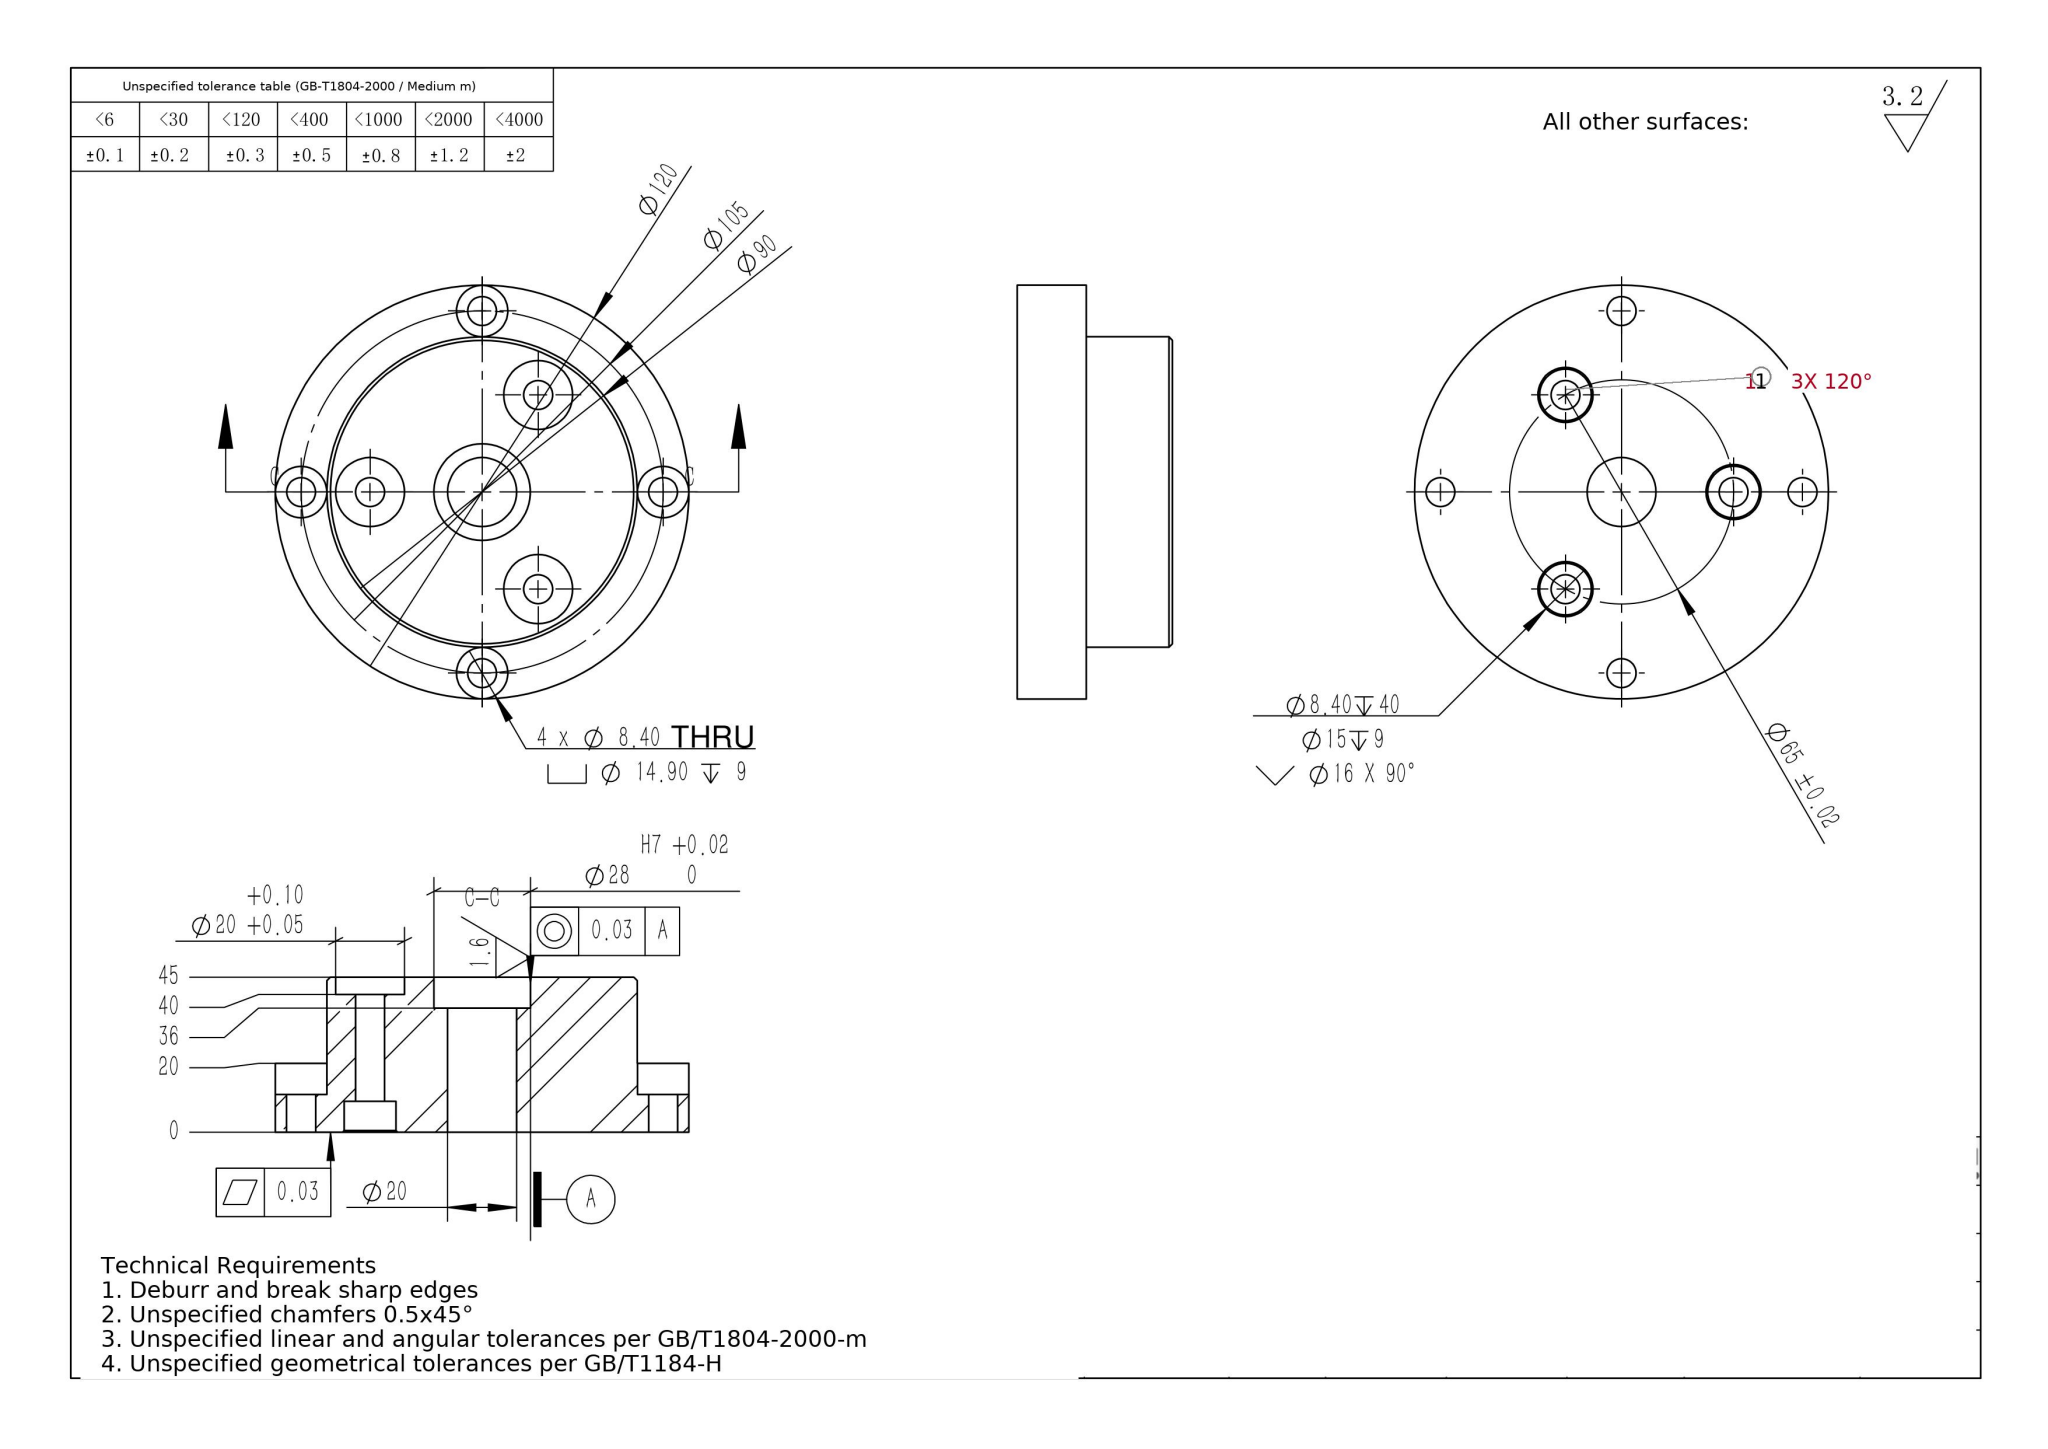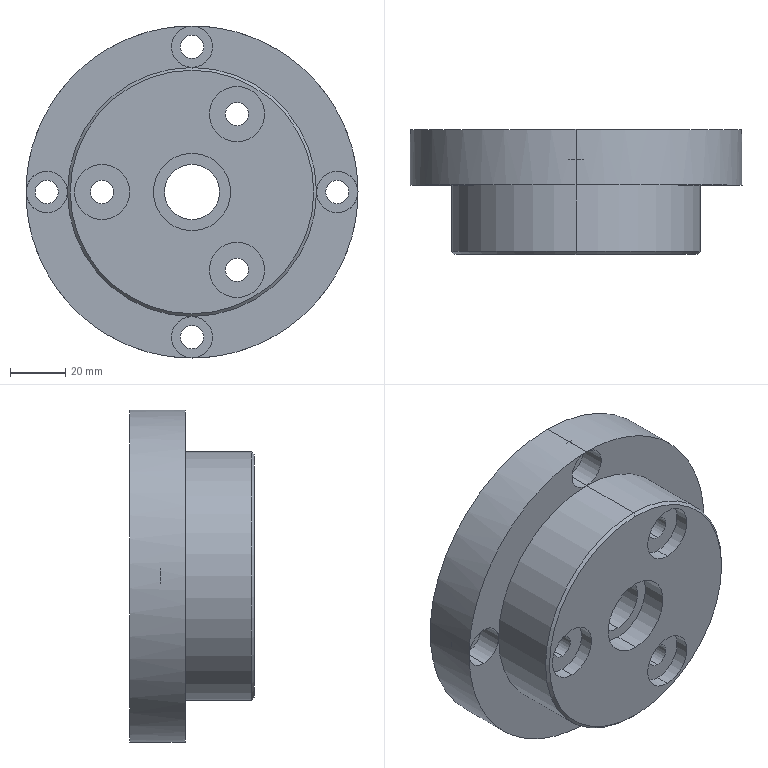Part | SolidWorks | mm | 1 solid | 64 faces | box 120 x 45 x 120 mm | volume 344875 mm3 | cylinder 42 | plane 14 | cone 8 | commonest cylinder face diameters 8.4 x14 20 x8 14.9 x8 15 x6 28 x2 90 x2 120 x2
build123d program:
from build123d import *

# Parameters (mm, degrees)
SKETCH1_W                                         = 60
SKETCH1_H                                         = 20
SKETCH2_R                                         = 45
BOSS_EXTRUDE1_DEPTH                               = 25
HOLE_SIZE_ACCORDING_TO_HEXAGON_SOCKET_D           = 8.4
HOLE_SIZE_ACCORDING_TO_HEXAGON_SOCKET_CBORE_D     = 14.9
HOLE_SIZE_ACCORDING_TO_HEXAGON_SOCKET_CBORE_DEPTH = 9
HOLE_SIZE_ACCORDING_TO_HEXAGON_SO_2_D             = 8.4
HOLE_SIZE_ACCORDING_TO_HEXAGON_SO_2_CBORE_D       = 15
HOLE_SIZE_ACCORDING_TO_HEXAGON_SO_2_CBORE_DEPTH   = 9
CHAMFER1_SIZE                                     = 0.4998
CHAMFER1_SIZE2                                    = 0.4998
CHAMFER2_SIZE                                     = 1
CHAMFER2_SIZE2                                    = 1
SKETCH7_R                                         = 10
CUT_EXTRUDE1_DEPTH                                = 5
SKETCH8_R                                         = 14
CUT_EXTRUDE2_DEPTH                                = 9
SKETCH9_R                                         = 10
CUT_EXTRUDE3_DEPTH                                = 93.174


with BuildPart() as part:
    # Sketch1 → Revolve1 (revolve)
    with BuildSketch(Plane(origin=(0, 0, 0), x_dir=(-1, 0, 0), z_dir=(0, 0, -1)), mode=Mode.PRIVATE) as revolve1_sk:
        with Locations((-30, 12.5)):
            Rectangle(SKETCH1_W, SKETCH1_H)
    revolve(revolve1_sk.sketch.rotate(Axis((0, 2.5, 0), (0, 1, 0)), 270), axis=Axis((0, 2.5, 0), (0, 1, 0)))

    # Sketch2 → Boss-Extrude1 (add)
    with BuildSketch(Plane.XZ.offset(-2.5)):
        with Locations(Location((0, 0, 0), (0, 0, 90))):
            Circle(SKETCH2_R)
    extrude(amount=BOSS_EXTRUDE1_DEPTH)

    # Hole Size _ according to_ Hexagon Socket (through all)
    with Locations(Plane(origin=(0, 2.5, 0), x_dir=(-1, 0, 0), z_dir=(0, -1, 0))):
        with Locations((0, 52.5), (52.5, 0), (0, -52.5), (-52.5, 0)):
            CounterBoreHole(HOLE_SIZE_ACCORDING_TO_HEXAGON_SOCKET_D / 2, HOLE_SIZE_ACCORDING_TO_HEXAGON_SOCKET_CBORE_D / 2, HOLE_SIZE_ACCORDING_TO_HEXAGON_SOCKET_CBORE_DEPTH)

    # Hole Size _ according to_ Hexagon So 2 (through all)
    with Locations(Plane(origin=(0, 22.5, 0), x_dir=(1, 0, 0), z_dir=(0, 1, 0))):
        with Locations((16.25, -28.146), (16.25, 28.146), (-32.5, 0)):
            CounterBoreHole(HOLE_SIZE_ACCORDING_TO_HEXAGON_SO_2_D / 2, HOLE_SIZE_ACCORDING_TO_HEXAGON_SO_2_CBORE_D / 2, HOLE_SIZE_ACCORDING_TO_HEXAGON_SO_2_CBORE_DEPTH)

    # Chamfer1
    chamfer1_edges = [part.edges().sort_by_distance(p)[0] for p in [
        (-40, 22.5, 0),
        (8.75, 22.5, -28.146),
        (8.75, 22.5, 28.146),
    ]]
    chamfer1_side = [part.faces().sort_by_distance(p)[0] for p in [
        (0, 22.5, 0),
    ]]
    chamfer(chamfer1_edges, length=CHAMFER1_SIZE, length2=CHAMFER1_SIZE2, reference=chamfer1_side[0])

    # Chamfer2
    chamfer2_edges = [part.edges().sort_by_distance(p)[0] for p in [
        (0, -22.5, -45),
    ]]
    chamfer2_side = [part.faces().sort_by_distance(p)[0] for p in [
        (0, -10, -45),
    ]]
    chamfer(chamfer2_edges, length=CHAMFER2_SIZE, length2=CHAMFER2_SIZE2, reference=chamfer2_side[0])

    # Sketch7 → Cut-Extrude1 (cut)
    with BuildSketch(Plane.XZ.offset(22.5)):
        with Locations(Location((-32.5, 0, 0), (0, 0, 270))):
            Circle(SKETCH7_R)
        with Locations(Location((16.25, 28.146, 0), (0, 0, 270))):
            Circle(SKETCH7_R)
        with Locations(Location((16.25, -28.146, 0), (0, 0, 270))):
            Circle(SKETCH7_R)
    extrude(amount=-CUT_EXTRUDE1_DEPTH, mode=Mode.SUBTRACT)

    # Sketch8 → Cut-Extrude2 (cut)
    with BuildSketch(Plane.XZ.offset(22.5)):
        with Locations(Location((0, 0, 0), (0, 0, 270))):
            Circle(SKETCH8_R)
    extrude(amount=-CUT_EXTRUDE2_DEPTH, mode=Mode.SUBTRACT)

    # Sketch9 → Cut-Extrude3 (cut, through all)
    with BuildSketch(Plane.XZ.offset(13.5)):
        with Locations(Location((0, 0, 0), (0, 0, 270))):
            Circle(SKETCH9_R)
    extrude(amount=-CUT_EXTRUDE3_DEPTH, mode=Mode.SUBTRACT)


solid = part.part